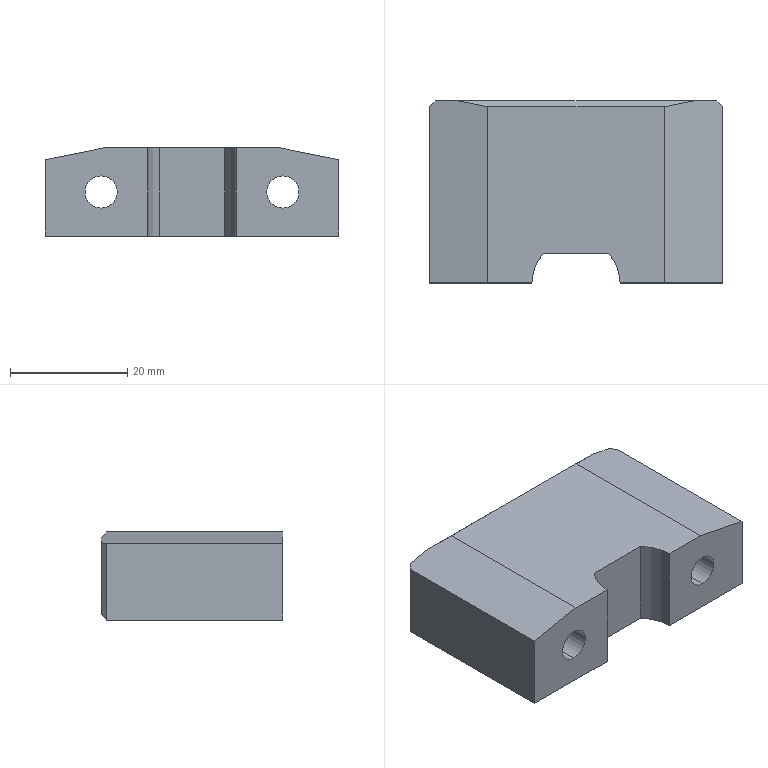Component | SolidWorks | XT-1-18-2-1 | 1 solid | 26 faces | box 50 x 31 x 15 mm | volume 18972 mm3 | plane 16 | cylinder 10 | commonest cylinder face diameters 10 x4 5.5 x4 15 x2
build123d program:
from build123d import *

# Parameters (mm, degrees)
BOSS_EXTRUDE1_DEPTH                             = 15
M5_HEX_SOCKET_HEAD_CAP_SCREW_CBORE1_D           = 5.5
M5_HEX_SOCKET_HEAD_CAP_SCREW_CBORE1_CBORE_D     = 10
M5_HEX_SOCKET_HEAD_CAP_SCREW_CBORE1_CBORE_DEPTH = 10
CHAMFER1_SIZE                                   = 10
CHAMFER1_SIZE2                                  = 2
CHAMFER2_SIZE                                   = 1
CHAMFER3_SIZE                                   = 1


with BuildPart() as part:
    # Sketch1 → Boss-Extrude1 (new body)
    with BuildSketch(Plane.XY):
        with BuildLine():
            Line((19.41, -26), (30.59, -26))
            ThreePointArc((30.59, -26), (32.006, -28.324), (32.5, -31))
            Line((32.5, -31), (50, -31))
            Line((50, -31), (50, 0))
            Line((50, 0), (0, 0))
            Line((0, 0), (0, -31))
            Line((0, -31), (17.5, -31))
            ThreePointArc((17.5, -31), (17.994, -28.324), (19.41, -26))
        make_face()
    extrude(amount=BOSS_EXTRUDE1_DEPTH)

    # M5 Hex Socket Head Cap Screw CBORE1 (through all)
    with Locations(Plane(origin=(0, 0, 0), x_dir=(1, 0, 0), z_dir=(0, 1, 0))):
        with Locations((9.5, -7.5), (40.5, -7.5)):
            CounterBoreHole(M5_HEX_SOCKET_HEAD_CAP_SCREW_CBORE1_D / 2, M5_HEX_SOCKET_HEAD_CAP_SCREW_CBORE1_CBORE_D / 2, M5_HEX_SOCKET_HEAD_CAP_SCREW_CBORE1_CBORE_DEPTH)

    # Chamfer1
    chamfer1_edges = [part.edges().sort_by_distance(p)[0] for p in [
        (0, -15.5, 0),
        (50, -15.5, 0),
    ]]
    chamfer1_side = [part.faces().sort_by_distance(p)[0] for p in [
        (25, -14.889, 0),
    ]]
    chamfer(chamfer1_edges, length=CHAMFER1_SIZE, length2=CHAMFER1_SIZE2, reference=chamfer1_side[0])

    # Chamfer2
    chamfer2_edges = [part.edges().sort_by_distance(p)[0] for p in [
        (25, 0, 15),
        (25, 0, 0),
    ]]
    chamfer(chamfer2_edges, length=CHAMFER2_SIZE)

    # Chamfer3
    chamfer3_edges = [part.edges().sort_by_distance(p)[0] for p in [
        (0, 0, 8),
        (50, 0, 8),
    ]]
    chamfer(chamfer3_edges, length=CHAMFER3_SIZE)


solid = part.part

# Placed as in the assembly
solid = solid.moved(Location((964.283, 139.385, -138), (-180, 0, 180)))
STEP:
#1=CARTESIAN_POINT('',(37.59,5.094,-5.531));
#2=VERTEX_POINT('',#1);
#3=CARTESIAN_POINT('',(37.59,5.094,-5.925));
#4=VERTEX_POINT('',#3);
#5=CARTESIAN_POINT('',(37.59,5.094,-5.728));
#6=DIRECTION('',(0.,1.,0.));
#7=DIRECTION('',(0.,0.,-1.));
#8=AXIS2_PLACEMENT_3D('',#5,#6,#7);
#9=CIRCLE('',#8,0.1969);
#10=EDGE_CURVE('',#2,#4,#9,.T.);
#11=ORIENTED_EDGE('',*,*,#10,.F.);
#12=CARTESIAN_POINT('',(37.59,5.488,-5.531));
#13=VERTEX_POINT('',#12);
#14=CARTESIAN_POINT('',(37.59,5.488,-5.531));
#15=DIRECTION('',(0.,1.,0.));
#16=VECTOR('',#15,39.37);
#17=LINE('',#14,#16);
#18=EDGE_CURVE('',#2,#13,#17,.T.);
#19=ORIENTED_EDGE('',*,*,#18,.T.);
#20=CARTESIAN_POINT('',(37.59,5.488,-5.925));
#21=VERTEX_POINT('',#20);
#22=CARTESIAN_POINT('',(37.59,5.488,-5.728));
#23=DIRECTION('',(0.,1.,0.));
#24=DIRECTION('',(0.,0.,-1.));
#25=AXIS2_PLACEMENT_3D('',#22,#23,#24);
#26=CIRCLE('',#25,0.1969);
#27=EDGE_CURVE('',#13,#21,#26,.T.);
#28=ORIENTED_EDGE('',*,*,#27,.T.);
#29=CARTESIAN_POINT('',(37.59,5.488,-5.925));
#30=DIRECTION('',(0.,1.,0.));
#31=VECTOR('',#30,39.37);
#32=LINE('',#29,#31);
#33=EDGE_CURVE('',#4,#21,#32,.T.);
#34=ORIENTED_EDGE('',*,*,#33,.F.);
#35=EDGE_LOOP('',(#11,#19,#28,#34));
#36=FACE_OUTER_BOUND('',#35,.T.);
#37=CARTESIAN_POINT('',(37.59,5.488,-5.728));
#38=DIRECTION('',(0.,1.,0.));
#39=DIRECTION('',(0.,0.,-1.));
#40=AXIS2_PLACEMENT_3D('',#37,#38,#39);
#41=CYLINDRICAL_SURFACE('',#40,0.1969);
#42=ADVANCED_FACE('',(#36),#41,.F.);
#43=CARTESIAN_POINT('',(37.59,4.267,-5.62));
#44=VERTEX_POINT('',#43);
#45=CARTESIAN_POINT('',(37.59,4.267,-5.837));
#46=VERTEX_POINT('',#45);
#47=CARTESIAN_POINT('',(37.59,4.267,-5.728));
#48=DIRECTION('',(0.,1.,0.));
#49=DIRECTION('',(0.,0.,-1.));
#50=AXIS2_PLACEMENT_3D('',#47,#48,#49);
#51=CIRCLE('',#50,0.1083);
#52=EDGE_CURVE('',#44,#46,#51,.T.);
#53=ORIENTED_EDGE('',*,*,#52,.F.);
#54=CARTESIAN_POINT('',(37.59,5.094,-5.62));
#55=VERTEX_POINT('',#54);
#56=CARTESIAN_POINT('',(37.59,5.488,-5.62));
#57=DIRECTION('',(0.,1.,0.));
#58=VECTOR('',#57,39.37);
#59=LINE('',#56,#58);
#60=EDGE_CURVE('',#44,#55,#59,.T.);
#61=ORIENTED_EDGE('',*,*,#60,.T.);
#62=CARTESIAN_POINT('',(37.59,5.094,-5.837));
#63=VERTEX_POINT('',#62);
#64=CARTESIAN_POINT('',(37.59,5.094,-5.728));
#65=DIRECTION('',(0.,1.,0.));
#66=DIRECTION('',(0.,0.,-1.));
#67=AXIS2_PLACEMENT_3D('',#64,#65,#66);
#68=CIRCLE('',#67,0.1083);
#69=EDGE_CURVE('',#55,#63,#68,.T.);
#70=ORIENTED_EDGE('',*,*,#69,.T.);
#71=CARTESIAN_POINT('',(37.59,5.488,-5.837));
#72=DIRECTION('',(0.,1.,0.));
#73=VECTOR('',#72,39.37);
#74=LINE('',#71,#73);
#75=EDGE_CURVE('',#46,#63,#74,.T.);
#76=ORIENTED_EDGE('',*,*,#75,.F.);
#77=EDGE_LOOP('',(#53,#61,#70,#76));
#78=FACE_OUTER_BOUND('',#77,.T.);
#79=CARTESIAN_POINT('',(37.59,5.488,-5.728));
#80=DIRECTION('',(0.,1.,0.));
#81=DIRECTION('',(0.,0.,-1.));
#82=AXIS2_PLACEMENT_3D('',#79,#80,#81);
#83=CYLINDRICAL_SURFACE('',#82,0.1083);
#84=ADVANCED_FACE('',(#78),#83,.F.);
#85=CARTESIAN_POINT('',(36.369,5.094,-5.531));
#86=VERTEX_POINT('',#85);
#87=CARTESIAN_POINT('',(36.369,5.094,-5.925));
#88=VERTEX_POINT('',#87);
#89=CARTESIAN_POINT('',(36.369,5.094,-5.728));
#90=DIRECTION('',(0.,1.,0.));
#91=DIRECTION('',(0.,0.,-1.));
#92=AXIS2_PLACEMENT_3D('',#89,#90,#91);
#93=CIRCLE('',#92,0.1969);
#94=EDGE_CURVE('',#86,#88,#93,.T.);
#95=ORIENTED_EDGE('',*,*,#94,.F.);
#96=CARTESIAN_POINT('',(36.369,5.488,-5.531));
#97=VERTEX_POINT('',#96);
#98=CARTESIAN_POINT('',(36.369,5.488,-5.531));
#99=DIRECTION('',(0.,1.,0.));
#100=VECTOR('',#99,39.37);
#101=LINE('',#98,#100);
#102=EDGE_CURVE('',#86,#97,#101,.T.);
#103=ORIENTED_EDGE('',*,*,#102,.T.);
#104=CARTESIAN_POINT('',(36.369,5.488,-5.925));
#105=VERTEX_POINT('',#104);
#106=CARTESIAN_POINT('',(36.369,5.488,-5.728));
#107=DIRECTION('',(0.,1.,0.));
#108=DIRECTION('',(0.,0.,-1.));
#109=AXIS2_PLACEMENT_3D('',#106,#107,#108);
#110=CIRCLE('',#109,0.1969);
#111=EDGE_CURVE('',#97,#105,#110,.T.);
#112=ORIENTED_EDGE('',*,*,#111,.T.);
#113=CARTESIAN_POINT('',(36.369,5.488,-5.925));
#114=DIRECTION('',(0.,1.,0.));
#115=VECTOR('',#114,39.37);
#116=LINE('',#113,#115);
#117=EDGE_CURVE('',#88,#105,#116,.T.);
#118=ORIENTED_EDGE('',*,*,#117,.F.);
#119=EDGE_LOOP('',(#95,#103,#112,#118));
#120=FACE_OUTER_BOUND('',#119,.T.);
#121=CARTESIAN_POINT('',(36.369,5.488,-5.728));
#122=DIRECTION('',(0.,1.,0.));
#123=DIRECTION('',(0.,0.,-1.));
#124=AXIS2_PLACEMENT_3D('',#121,#122,#123);
#125=CYLINDRICAL_SURFACE('',#124,0.1969);
#126=ADVANCED_FACE('',(#120),#125,.F.);
#127=CARTESIAN_POINT('',(36.369,4.267,-5.62));
#128=VERTEX_POINT('',#127);
#129=CARTESIAN_POINT('',(36.369,4.267,-5.837));
#130=VERTEX_POINT('',#129);
#131=CARTESIAN_POINT('',(36.369,4.267,-5.728));
#132=DIRECTION('',(0.,1.,0.));
#133=DIRECTION('',(0.,0.,-1.));
#134=AXIS2_PLACEMENT_3D('',#131,#132,#133);
#135=CIRCLE('',#134,0.1083);
#136=EDGE_CURVE('',#128,#130,#135,.T.);
#137=ORIENTED_EDGE('',*,*,#136,.F.);
#138=CARTESIAN_POINT('',(36.369,5.094,-5.62));
#139=VERTEX_POINT('',#138);
#140=CARTESIAN_POINT('',(36.369,5.488,-5.62));
#141=DIRECTION('',(0.,1.,0.));
#142=VECTOR('',#141,39.37);
#143=LINE('',#140,#142);
#144=EDGE_CURVE('',#128,#139,#143,.T.);
#145=ORIENTED_EDGE('',*,*,#144,.T.);
#146=CARTESIAN_POINT('',(36.369,5.094,-5.837));
#147=VERTEX_POINT('',#146);
#148=CARTESIAN_POINT('',(36.369,5.094,-5.728));
#149=DIRECTION('',(0.,1.,0.));
#150=DIRECTION('',(0.,0.,-1.));
#151=AXIS2_PLACEMENT_3D('',#148,#149,#150);
#152=CIRCLE('',#151,0.1083);
#153=EDGE_CURVE('',#139,#147,#152,.T.);
#154=ORIENTED_EDGE('',*,*,#153,.T.);
#155=CARTESIAN_POINT('',(36.369,5.488,-5.837));
#156=DIRECTION('',(0.,1.,0.));
#157=VECTOR('',#156,39.37);
#158=LINE('',#155,#157);
#159=EDGE_CURVE('',#130,#147,#158,.T.);
#160=ORIENTED_EDGE('',*,*,#159,.F.);
#161=EDGE_LOOP('',(#137,#145,#154,#160));
#162=FACE_OUTER_BOUND('',#161,.T.);
#163=CARTESIAN_POINT('',(36.369,5.488,-5.728));
#164=DIRECTION('',(0.,1.,0.));
#165=DIRECTION('',(0.,0.,-1.));
#166=AXIS2_PLACEMENT_3D('',#163,#164,#165);
#167=CYLINDRICAL_SURFACE('',#166,0.1083);
#168=ADVANCED_FACE('',(#162),#167,.F.);
#169=CARTESIAN_POINT('',(37.964,5.448,-6.024));
#170=VERTEX_POINT('',#169);
#171=CARTESIAN_POINT('',(37.964,4.267,-6.024));
#172=VERTEX_POINT('',#171);
#173=CARTESIAN_POINT('',(37.964,5.488,-6.024));
#174=DIRECTION('',(-0.,-1.,0.));
#175=VECTOR('',#174,39.37);
#176=LINE('',#173,#175);
#177=EDGE_CURVE('',#170,#172,#176,.T.);
#178=ORIENTED_EDGE('',*,*,#177,.F.);
#179=CARTESIAN_POINT('',(37.964,5.448,-5.512));
#180=VERTEX_POINT('',#179);
#181=CARTESIAN_POINT('',(37.964,5.448,-6.024));
#182=DIRECTION('',(0.,0.,1.));
#183=VECTOR('',#182,39.37);
#184=LINE('',#181,#183);
#185=EDGE_CURVE('',#170,#180,#184,.T.);
#186=ORIENTED_EDGE('',*,*,#185,.T.);
#187=CARTESIAN_POINT('',(37.964,4.267,-5.512));
#188=VERTEX_POINT('',#187);
#189=CARTESIAN_POINT('',(37.964,5.488,-5.512));
#190=DIRECTION('',(-0.,-1.,0.));
#191=VECTOR('',#190,39.37);
#192=LINE('',#189,#191);
#193=EDGE_CURVE('',#180,#188,#192,.T.);
#194=ORIENTED_EDGE('',*,*,#193,.T.);
#195=CARTESIAN_POINT('',(37.964,4.267,-6.024));
#196=DIRECTION('',(0.,0.,1.));
#197=VECTOR('',#196,39.37);
#198=LINE('',#195,#197);
#199=EDGE_CURVE('',#172,#188,#198,.T.);
#200=ORIENTED_EDGE('',*,*,#199,.F.);
#201=EDGE_LOOP('',(#178,#186,#194,#200));
#202=FACE_OUTER_BOUND('',#201,.T.);
#203=CARTESIAN_POINT('',(37.964,5.488,-6.024));
#204=DIRECTION('',(-1.,0.,0.));
#205=DIRECTION('',(0.,1.,0.));
#206=AXIS2_PLACEMENT_3D('',#203,#204,#205);
#207=PLANE('',#206);
#208=ADVANCED_FACE('',(#202),#207,.F.);
#209=CARTESIAN_POINT('',(37.59,4.267,-5.728));
#210=DIRECTION('',(0.,1.,0.));
#211=DIRECTION('',(0.,0.,-1.));
#212=AXIS2_PLACEMENT_3D('',#209,#210,#211);
#213=CIRCLE('',#212,0.1083);
#214=EDGE_CURVE('',#46,#44,#213,.T.);
#215=ORIENTED_EDGE('',*,*,#214,.T.);
#216=ORIENTED_EDGE('',*,*,#52,.T.);
#217=EDGE_LOOP('',(#215,#216));
#218=FACE_BOUND('',#217,.T.);
#219=ORIENTED_EDGE('',*,*,#199,.T.);
#220=CARTESIAN_POINT('',(37.57,4.267,-5.433));
#221=VERTEX_POINT('',#220);
#222=CARTESIAN_POINT('',(37.964,4.267,-5.512));
#223=DIRECTION('',(-0.9806,0.,0.1961));
#224=VECTOR('',#223,39.37);
#225=LINE('',#222,#224);
#226=EDGE_CURVE('',#188,#221,#225,.T.);
#227=ORIENTED_EDGE('',*,*,#226,.T.);
#228=CARTESIAN_POINT('',(37.275,4.267,-5.433));
#229=VERTEX_POINT('',#228);
#230=CARTESIAN_POINT('',(37.964,4.267,-5.433));
#231=DIRECTION('',(-1.,0.,0.));
#232=VECTOR('',#231,39.37);
#233=LINE('',#230,#232);
#234=EDGE_CURVE('',#221,#229,#233,.T.);
#235=ORIENTED_EDGE('',*,*,#234,.T.);
#236=CARTESIAN_POINT('',(37.275,4.267,-6.024));
#237=VERTEX_POINT('',#236);
#238=CARTESIAN_POINT('',(37.275,4.267,-6.024));
#239=DIRECTION('',(0.,0.,1.));
#240=VECTOR('',#239,39.37);
#241=LINE('',#238,#240);
#242=EDGE_CURVE('',#237,#229,#241,.T.);
#243=ORIENTED_EDGE('',*,*,#242,.F.);
#244=CARTESIAN_POINT('',(37.964,4.267,-6.024));
#245=DIRECTION('',(-1.,0.,0.));
#246=VECTOR('',#245,39.37);
#247=LINE('',#244,#246);
#248=EDGE_CURVE('',#172,#237,#247,.T.);
#249=ORIENTED_EDGE('',*,*,#248,.F.);
#250=EDGE_LOOP('',(#219,#227,#235,#243,#249));
#251=FACE_OUTER_BOUND('',#250,.T.);
#252=CARTESIAN_POINT('',(37.964,4.267,-6.024));
#253=DIRECTION('',(0.,1.,0.));
#254=DIRECTION('',(0.,0.,-1.));
#255=AXIS2_PLACEMENT_3D('',#252,#253,#254);
#256=PLANE('',#255);
#257=ADVANCED_FACE('',(#218,#251),#256,.F.);
#258=CARTESIAN_POINT('',(37.2,4.464,-5.433));
#259=VERTEX_POINT('',#258);
#260=CARTESIAN_POINT('',(36.98,4.267,-5.433));
#261=DIRECTION('',(0.,0.,1.));
#262=DIRECTION('',(-1.,0.,0.));
#263=AXIS2_PLACEMENT_3D('',#260,#261,#262);
#264=CIRCLE('',#263,0.2953);
#265=EDGE_CURVE('',#229,#259,#264,.T.);
#266=ORIENTED_EDGE('',*,*,#265,.T.);
#267=CARTESIAN_POINT('',(37.2,4.464,-6.024));
#268=VERTEX_POINT('',#267);
#269=CARTESIAN_POINT('',(37.2,4.464,-6.024));
#270=DIRECTION('',(0.,0.,1.));
#271=VECTOR('',#270,39.37);
#272=LINE('',#269,#271);
#273=EDGE_CURVE('',#268,#259,#272,.T.);
#274=ORIENTED_EDGE('',*,*,#273,.F.);
#275=CARTESIAN_POINT('',(36.98,4.267,-6.024));
#276=DIRECTION('',(0.,0.,1.));
#277=DIRECTION('',(-1.,0.,0.));
#278=AXIS2_PLACEMENT_3D('',#275,#276,#277);
#279=CIRCLE('',#278,0.2953);
#280=EDGE_CURVE('',#237,#268,#279,.T.);
#281=ORIENTED_EDGE('',*,*,#280,.F.);
#282=ORIENTED_EDGE('',*,*,#242,.T.);
#283=EDGE_LOOP('',(#266,#274,#281,#282));
#284=FACE_OUTER_BOUND('',#283,.T.);
#285=CARTESIAN_POINT('',(36.98,4.267,-6.024));
#286=DIRECTION('',(0.,0.,1.));
#287=DIRECTION('',(1.,0.,0.));
#288=AXIS2_PLACEMENT_3D('',#285,#286,#287);
#289=CYLINDRICAL_SURFACE('',#288,0.2953);
#290=ADVANCED_FACE('',(#284),#289,.F.);
#291=CARTESIAN_POINT('',(36.76,4.464,-5.433));
#292=VERTEX_POINT('',#291);
#293=CARTESIAN_POINT('',(37.2,4.464,-5.433));
#294=DIRECTION('',(-1.,0.,0.));
#295=VECTOR('',#294,39.37);
#296=LINE('',#293,#295);
#297=EDGE_CURVE('',#259,#292,#296,.T.);
#298=ORIENTED_EDGE('',*,*,#297,.T.);
#299=CARTESIAN_POINT('',(36.76,4.464,-6.024));
#300=VERTEX_POINT('',#299);
#301=CARTESIAN_POINT('',(36.76,4.464,-6.024));
#302=DIRECTION('',(0.,0.,1.));
#303=VECTOR('',#302,39.37);
#304=LINE('',#301,#303);
#305=EDGE_CURVE('',#300,#292,#304,.T.);
#306=ORIENTED_EDGE('',*,*,#305,.F.);
#307=CARTESIAN_POINT('',(37.2,4.464,-6.024));
#308=DIRECTION('',(-1.,0.,0.));
#309=VECTOR('',#308,39.37);
#310=LINE('',#307,#309);
#311=EDGE_CURVE('',#268,#300,#310,.T.);
#312=ORIENTED_EDGE('',*,*,#311,.F.);
#313=ORIENTED_EDGE('',*,*,#273,.T.);
#314=EDGE_LOOP('',(#298,#306,#312,#313));
#315=FACE_OUTER_BOUND('',#314,.T.);
#316=CARTESIAN_POINT('',(37.2,4.464,-6.024));
#317=DIRECTION('',(0.,1.,0.));
#318=DIRECTION('',(0.,0.,-1.));
#319=AXIS2_PLACEMENT_3D('',#316,#317,#318);
#320=PLANE('',#319);
#321=ADVANCED_FACE('',(#315),#320,.F.);
#322=CARTESIAN_POINT('',(36.684,4.267,-5.433));
#323=VERTEX_POINT('',#322);
#324=CARTESIAN_POINT('',(36.98,4.267,-5.433));
#325=DIRECTION('',(0.,0.,1.));
#326=DIRECTION('',(-1.,0.,0.));
#327=AXIS2_PLACEMENT_3D('',#324,#325,#326);
#328=CIRCLE('',#327,0.2953);
#329=EDGE_CURVE('',#292,#323,#328,.T.);
#330=ORIENTED_EDGE('',*,*,#329,.T.);
#331=CARTESIAN_POINT('',(36.684,4.267,-6.024));
#332=VERTEX_POINT('',#331);
#333=CARTESIAN_POINT('',(36.684,4.267,-6.024));
#334=DIRECTION('',(0.,0.,1.));
#335=VECTOR('',#334,39.37);
#336=LINE('',#333,#335);
#337=EDGE_CURVE('',#332,#323,#336,.T.);
#338=ORIENTED_EDGE('',*,*,#337,.F.);
#339=CARTESIAN_POINT('',(36.98,4.267,-6.024));
#340=DIRECTION('',(0.,0.,1.));
#341=DIRECTION('',(-1.,0.,0.));
#342=AXIS2_PLACEMENT_3D('',#339,#340,#341);
#343=CIRCLE('',#342,0.2953);
#344=EDGE_CURVE('',#300,#332,#343,.T.);
#345=ORIENTED_EDGE('',*,*,#344,.F.);
#346=ORIENTED_EDGE('',*,*,#305,.T.);
#347=EDGE_LOOP('',(#330,#338,#345,#346));
#348=FACE_OUTER_BOUND('',#347,.T.);
#349=CARTESIAN_POINT('',(36.98,4.267,-6.024));
#350=DIRECTION('',(0.,0.,1.));
#351=DIRECTION('',(1.,0.,0.));
#352=AXIS2_PLACEMENT_3D('',#349,#350,#351);
#353=CYLINDRICAL_SURFACE('',#352,0.2953);
#354=ADVANCED_FACE('',(#348),#353,.F.);
#355=CARTESIAN_POINT('',(36.369,4.267,-5.728));
#356=DIRECTION('',(0.,1.,0.));
#357=DIRECTION('',(0.,0.,-1.));
#358=AXIS2_PLACEMENT_3D('',#355,#356,#357);
#359=CIRCLE('',#358,0.1083);
#360=EDGE_CURVE('',#130,#128,#359,.T.);
#361=ORIENTED_EDGE('',*,*,#360,.T.);
#362=ORIENTED_EDGE('',*,*,#136,.T.);
#363=EDGE_LOOP('',(#361,#362));
#364=FACE_BOUND('',#363,.T.);
#365=CARTESIAN_POINT('',(36.389,4.267,-5.433));
#366=VERTEX_POINT('',#365);
#367=CARTESIAN_POINT('',(36.684,4.267,-5.433));
#368=DIRECTION('',(-1.,0.,0.));
#369=VECTOR('',#368,39.37);
#370=LINE('',#367,#369);
#371=EDGE_CURVE('',#323,#366,#370,.T.);
#372=ORIENTED_EDGE('',*,*,#371,.T.);
#373=CARTESIAN_POINT('',(35.995,4.267,-5.512));
#374=VERTEX_POINT('',#373);
#375=CARTESIAN_POINT('',(35.995,4.267,-5.512));
#376=DIRECTION('',(-0.9806,0.,-0.1961));
#377=VECTOR('',#376,39.37);
#378=LINE('',#375,#377);
#379=EDGE_CURVE('',#366,#374,#378,.T.);
#380=ORIENTED_EDGE('',*,*,#379,.T.);
#381=CARTESIAN_POINT('',(35.995,4.267,-6.024));
#382=VERTEX_POINT('',#381);
#383=CARTESIAN_POINT('',(35.995,4.267,-6.024));
#384=DIRECTION('',(0.,0.,1.));
#385=VECTOR('',#384,39.37);
#386=LINE('',#383,#385);
#387=EDGE_CURVE('',#382,#374,#386,.T.);
#388=ORIENTED_EDGE('',*,*,#387,.F.);
#389=CARTESIAN_POINT('',(36.684,4.267,-6.024));
#390=DIRECTION('',(-1.,0.,0.));
#391=VECTOR('',#390,39.37);
#392=LINE('',#389,#391);
#393=EDGE_CURVE('',#332,#382,#392,.T.);
#394=ORIENTED_EDGE('',*,*,#393,.F.);
#395=ORIENTED_EDGE('',*,*,#337,.T.);
#396=EDGE_LOOP('',(#372,#380,#388,#394,#395));
#397=FACE_OUTER_BOUND('',#396,.T.);
#398=CARTESIAN_POINT('',(36.684,4.267,-6.024));
#399=DIRECTION('',(0.,1.,0.));
#400=DIRECTION('',(1.,-0.,0.));
#401=AXIS2_PLACEMENT_3D('',#398,#399,#400);
#402=PLANE('',#401);
#403=ADVANCED_FACE('',(#364,#397),#402,.F.);
#404=CARTESIAN_POINT('',(35.995,5.448,-5.512));
#405=VERTEX_POINT('',#404);
#406=CARTESIAN_POINT('',(35.995,5.488,-5.512));
#407=DIRECTION('',(0.,1.,0.));
#408=VECTOR('',#407,39.37);
#409=LINE('',#406,#408);
#410=EDGE_CURVE('',#374,#405,#409,.T.);
#411=ORIENTED_EDGE('',*,*,#410,.T.);
#412=CARTESIAN_POINT('',(35.995,5.448,-6.024));
#413=VERTEX_POINT('',#412);
#414=CARTESIAN_POINT('',(35.995,5.448,-6.024));
#415=DIRECTION('',(0.,0.,-1.));
#416=VECTOR('',#415,39.37);
#417=LINE('',#414,#416);
#418=EDGE_CURVE('',#405,#413,#417,.T.);
#419=ORIENTED_EDGE('',*,*,#418,.T.);
#420=CARTESIAN_POINT('',(35.995,5.488,-6.024));
#421=DIRECTION('',(0.,1.,0.));
#422=VECTOR('',#421,39.37);
#423=LINE('',#420,#422);
#424=EDGE_CURVE('',#382,#413,#423,.T.);
#425=ORIENTED_EDGE('',*,*,#424,.F.);
#426=ORIENTED_EDGE('',*,*,#387,.T.);
#427=EDGE_LOOP('',(#411,#419,#425,#426));
#428=FACE_OUTER_BOUND('',#427,.T.);
#429=CARTESIAN_POINT('',(35.995,5.488,-6.024));
#430=DIRECTION('',(1.,-0.,0.));
#431=DIRECTION('',(-0.,-1.,0.));
#432=AXIS2_PLACEMENT_3D('',#429,#430,#431);
#433=PLANE('',#432);
#434=ADVANCED_FACE('',(#428),#433,.F.);
#435=CARTESIAN_POINT('',(37.59,5.488,-5.728));
#436=DIRECTION('',(0.,1.,0.));
#437=DIRECTION('',(0.,0.,-1.));
#438=AXIS2_PLACEMENT_3D('',#435,#436,#437);
#439=CIRCLE('',#438,0.1969);
#440=EDGE_CURVE('',#21,#13,#439,.T.);
#441=ORIENTED_EDGE('',*,*,#440,.F.);
#442=ORIENTED_EDGE('',*,*,#27,.F.);
#443=EDGE_LOOP('',(#441,#442));
#444=FACE_BOUND('',#443,.T.);
#445=CARTESIAN_POINT('',(36.369,5.488,-5.728));
#446=DIRECTION('',(0.,1.,0.));
#447=DIRECTION('',(0.,0.,-1.));
#448=AXIS2_PLACEMENT_3D('',#445,#446,#447);
#449=CIRCLE('',#448,0.1969);
#450=EDGE_CURVE('',#105,#97,#449,.T.);
#451=ORIENTED_EDGE('',*,*,#450,.F.);
#452=ORIENTED_EDGE('',*,*,#111,.F.);
#453=EDGE_LOOP('',(#451,#452));
#454=FACE_BOUND('',#453,.T.);
#455=CARTESIAN_POINT('',(37.767,5.488,-5.472));
#456=VERTEX_POINT('',#455);
#457=CARTESIAN_POINT('',(37.925,5.488,-5.504));
#458=VERTEX_POINT('',#457);
#459=CARTESIAN_POINT('',(37.964,5.488,-5.512));
#460=DIRECTION('',(0.9806,0.,-0.1961));
#461=VECTOR('',#460,39.37);
#462=LINE('',#459,#461);
#463=EDGE_CURVE('',#456,#458,#462,.T.);
#464=ORIENTED_EDGE('',*,*,#463,.T.);
#465=CARTESIAN_POINT('',(37.925,5.488,-5.984));
#466=VERTEX_POINT('',#465);
#467=CARTESIAN_POINT('',(37.925,5.488,-6.024));
#468=DIRECTION('',(0.,0.,-1.));
#469=VECTOR('',#468,39.37);
#470=LINE('',#467,#469);
#471=EDGE_CURVE('',#458,#466,#470,.T.);
#472=ORIENTED_EDGE('',*,*,#471,.T.);
#473=CARTESIAN_POINT('',(36.035,5.488,-5.984));
#474=VERTEX_POINT('',#473);
#475=CARTESIAN_POINT('',(35.995,5.488,-5.984));
#476=DIRECTION('',(-1.,0.,0.));
#477=VECTOR('',#476,39.37);
#478=LINE('',#475,#477);
#479=EDGE_CURVE('',#466,#474,#478,.T.);
#480=ORIENTED_EDGE('',*,*,#479,.T.);
#481=CARTESIAN_POINT('',(36.035,5.488,-5.504));
#482=VERTEX_POINT('',#481);
#483=CARTESIAN_POINT('',(36.035,5.488,-6.024));
#484=DIRECTION('',(0.,0.,1.));
#485=VECTOR('',#484,39.37);
#486=LINE('',#483,#485);
#487=EDGE_CURVE('',#474,#482,#486,.T.);
#488=ORIENTED_EDGE('',*,*,#487,.T.);
#489=CARTESIAN_POINT('',(36.192,5.488,-5.472));
#490=VERTEX_POINT('',#489);
#491=CARTESIAN_POINT('',(35.995,5.488,-5.512));
#492=DIRECTION('',(0.9806,0.,0.1961));
#493=VECTOR('',#492,39.37);
#494=LINE('',#491,#493);
#495=EDGE_CURVE('',#482,#490,#494,.T.);
#496=ORIENTED_EDGE('',*,*,#495,.T.);
#497=CARTESIAN_POINT('',(37.964,5.488,-5.472));
#498=DIRECTION('',(1.,0.,0.));
#499=VECTOR('',#498,39.37);
#500=LINE('',#497,#499);
#501=EDGE_CURVE('',#490,#456,#500,.T.);
#502=ORIENTED_EDGE('',*,*,#501,.T.);
#503=EDGE_LOOP('',(#464,#472,#480,#488,#496,#502));
#504=FACE_OUTER_BOUND('',#503,.T.);
#505=CARTESIAN_POINT('',(37.964,5.488,-6.024));
#506=DIRECTION('',(0.,-1.,0.));
#507=DIRECTION('',(0.,0.,1.));
#508=AXIS2_PLACEMENT_3D('',#505,#506,#507);
#509=PLANE('',#508);
#510=ADVANCED_FACE('',(#444,#454,#504),#509,.F.);
#511=ORIENTED_EDGE('',*,*,#424,.T.);
#512=CARTESIAN_POINT('',(37.964,5.448,-6.024));
#513=DIRECTION('',(1.,0.,0.));
#514=VECTOR('',#513,39.37);
#515=LINE('',#512,#514);
#516=EDGE_CURVE('',#413,#170,#515,.T.);
#517=ORIENTED_EDGE('',*,*,#516,.T.);
#518=ORIENTED_EDGE('',*,*,#177,.T.);
#519=ORIENTED_EDGE('',*,*,#248,.T.);
#520=ORIENTED_EDGE('',*,*,#280,.T.);
#521=ORIENTED_EDGE('',*,*,#311,.T.);
#522=ORIENTED_EDGE('',*,*,#344,.T.);
#523=ORIENTED_EDGE('',*,*,#393,.T.);
#524=EDGE_LOOP('',(#511,#517,#518,#519,#520,#521,#522,#523));
#525=FACE_OUTER_BOUND('',#524,.T.);
#526=CARTESIAN_POINT('',(36.98,4.267,-6.024));
#527=DIRECTION('',(0.,0.,-1.));
#528=DIRECTION('',(-1.,0.,0.));
#529=AXIS2_PLACEMENT_3D('',#526,#527,#528);
#530=PLANE('',#529);
#531=ADVANCED_FACE('',(#525),#530,.T.);
#532=CARTESIAN_POINT('',(37.57,5.448,-5.433));
#533=VERTEX_POINT('',#532);
#534=CARTESIAN_POINT('',(37.57,4.267,-5.433));
#535=DIRECTION('',(0.,1.,0.));
#536=VECTOR('',#535,39.37);
#537=LINE('',#534,#536);
#538=EDGE_CURVE('',#221,#533,#537,.T.);
#539=ORIENTED_EDGE('',*,*,#538,.T.);
#540=CARTESIAN_POINT('',(36.389,5.448,-5.433));
#541=VERTEX_POINT('',#540);
#542=CARTESIAN_POINT('',(36.98,5.448,-5.433));
#543=DIRECTION('',(-1.,0.,0.));
#544=VECTOR('',#543,39.37);
#545=LINE('',#542,#544);
#546=EDGE_CURVE('',#533,#541,#545,.T.);
#547=ORIENTED_EDGE('',*,*,#546,.T.);
#548=CARTESIAN_POINT('',(36.389,4.267,-5.433));
#549=DIRECTION('',(-0.,-1.,0.));
#550=VECTOR('',#549,39.37);
#551=LINE('',#548,#550);
#552=EDGE_CURVE('',#541,#366,#551,.T.);
#553=ORIENTED_EDGE('',*,*,#552,.T.);
#554=ORIENTED_EDGE('',*,*,#371,.F.);
#555=ORIENTED_EDGE('',*,*,#329,.F.);
#556=ORIENTED_EDGE('',*,*,#297,.F.);
#557=ORIENTED_EDGE('',*,*,#265,.F.);
#558=ORIENTED_EDGE('',*,*,#234,.F.);
#559=EDGE_LOOP('',(#539,#547,#553,#554,#555,#556,#557,#558));
#560=FACE_OUTER_BOUND('',#559,.T.);
#561=CARTESIAN_POINT('',(36.98,4.267,-5.433));
#562=DIRECTION('',(0.,0.,-1.));
#563=DIRECTION('',(-1.,0.,0.));
#564=AXIS2_PLACEMENT_3D('',#561,#562,#563);
#565=PLANE('',#564);
#566=ADVANCED_FACE('',(#560),#565,.F.);
#567=ORIENTED_EDGE('',*,*,#144,.F.);
#568=ORIENTED_EDGE('',*,*,#360,.F.);
#569=ORIENTED_EDGE('',*,*,#159,.T.);
#570=CARTESIAN_POINT('',(36.369,5.094,-5.728));
#571=DIRECTION('',(0.,1.,0.));
#572=DIRECTION('',(0.,0.,-1.));
#573=AXIS2_PLACEMENT_3D('',#570,#571,#572);
#574=CIRCLE('',#573,0.1083);
#575=EDGE_CURVE('',#147,#139,#574,.T.);
#576=ORIENTED_EDGE('',*,*,#575,.T.);
#577=EDGE_LOOP('',(#567,#568,#569,#576));
#578=FACE_OUTER_BOUND('',#577,.T.);
#579=CARTESIAN_POINT('',(36.369,5.488,-5.728));
#580=DIRECTION('',(0.,1.,0.));
#581=DIRECTION('',(0.,0.,-1.));
#582=AXIS2_PLACEMENT_3D('',#579,#580,#581);
#583=CYLINDRICAL_SURFACE('',#582,0.1083);
#584=ADVANCED_FACE('',(#578),#583,.F.);
#585=ORIENTED_EDGE('',*,*,#575,.F.);
#586=ORIENTED_EDGE('',*,*,#153,.F.);
#587=EDGE_LOOP('',(#585,#586));
#588=FACE_BOUND('',#587,.T.);
#589=CARTESIAN_POINT('',(36.369,5.094,-5.728));
#590=DIRECTION('',(0.,1.,0.));
#591=DIRECTION('',(0.,0.,-1.));
#592=AXIS2_PLACEMENT_3D('',#589,#590,#591);
#593=CIRCLE('',#592,0.1969);
#594=EDGE_CURVE('',#88,#86,#593,.T.);
#595=ORIENTED_EDGE('',*,*,#594,.T.);
#596=ORIENTED_EDGE('',*,*,#94,.T.);
#597=EDGE_LOOP('',(#595,#596));
#598=FACE_OUTER_BOUND('',#597,.T.);
#599=CARTESIAN_POINT('',(36.261,5.094,-5.728));
#600=DIRECTION('',(0.,-1.,0.));
#601=DIRECTION('',(0.,0.,1.));
#602=AXIS2_PLACEMENT_3D('',#599,#600,#601);
#603=PLANE('',#602);
#604=ADVANCED_FACE('',(#588,#598),#603,.F.);
#605=ORIENTED_EDGE('',*,*,#102,.F.);
#606=ORIENTED_EDGE('',*,*,#594,.F.);
#607=ORIENTED_EDGE('',*,*,#117,.T.);
#608=ORIENTED_EDGE('',*,*,#450,.T.);
#609=EDGE_LOOP('',(#605,#606,#607,#608));
#610=FACE_OUTER_BOUND('',#609,.T.);
#611=CARTESIAN_POINT('',(36.369,5.488,-5.728));
#612=DIRECTION('',(0.,1.,0.));
#613=DIRECTION('',(0.,0.,-1.));
#614=AXIS2_PLACEMENT_3D('',#611,#612,#613);
#615=CYLINDRICAL_SURFACE('',#614,0.1969);
#616=ADVANCED_FACE('',(#610),#615,.F.);
#617=ORIENTED_EDGE('',*,*,#60,.F.);
#618=ORIENTED_EDGE('',*,*,#214,.F.);
#619=ORIENTED_EDGE('',*,*,#75,.T.);
#620=CARTESIAN_POINT('',(37.59,5.094,-5.728));
#621=DIRECTION('',(0.,1.,0.));
#622=DIRECTION('',(0.,0.,-1.));
#623=AXIS2_PLACEMENT_3D('',#620,#621,#622);
#624=CIRCLE('',#623,0.1083);
#625=EDGE_CURVE('',#63,#55,#624,.T.);
#626=ORIENTED_EDGE('',*,*,#625,.T.);
#627=EDGE_LOOP('',(#617,#618,#619,#626));
#628=FACE_OUTER_BOUND('',#627,.T.);
#629=CARTESIAN_POINT('',(37.59,5.488,-5.728));
#630=DIRECTION('',(0.,1.,0.));
#631=DIRECTION('',(0.,0.,-1.));
#632=AXIS2_PLACEMENT_3D('',#629,#630,#631);
#633=CYLINDRICAL_SURFACE('',#632,0.1083);
#634=ADVANCED_FACE('',(#628),#633,.F.);
#635=ORIENTED_EDGE('',*,*,#625,.F.);
#636=ORIENTED_EDGE('',*,*,#69,.F.);
#637=EDGE_LOOP('',(#635,#636));
#638=FACE_BOUND('',#637,.T.);
#639=CARTESIAN_POINT('',(37.59,5.094,-5.728));
#640=DIRECTION('',(0.,1.,0.));
#641=DIRECTION('',(0.,0.,-1.));
#642=AXIS2_PLACEMENT_3D('',#639,#640,#641);
#643=CIRCLE('',#642,0.1969);
#644=EDGE_CURVE('',#4,#2,#643,.T.);
#645=ORIENTED_EDGE('',*,*,#644,.T.);
#646=ORIENTED_EDGE('',*,*,#10,.T.);
#647=EDGE_LOOP('',(#645,#646));
#648=FACE_OUTER_BOUND('',#647,.T.);
#649=CARTESIAN_POINT('',(37.482,5.094,-5.728));
#650=DIRECTION('',(0.,-1.,0.));
#651=DIRECTION('',(0.,0.,1.));
#652=AXIS2_PLACEMENT_3D('',#649,#650,#651);
#653=PLANE('',#652);
#654=ADVANCED_FACE('',(#638,#648),#653,.F.);
#655=ORIENTED_EDGE('',*,*,#18,.F.);
#656=ORIENTED_EDGE('',*,*,#644,.F.);
#657=ORIENTED_EDGE('',*,*,#33,.T.);
#658=ORIENTED_EDGE('',*,*,#440,.T.);
#659=EDGE_LOOP('',(#655,#656,#657,#658));
#660=FACE_OUTER_BOUND('',#659,.T.);
#661=CARTESIAN_POINT('',(37.59,5.488,-5.728));
#662=DIRECTION('',(0.,1.,0.));
#663=DIRECTION('',(0.,0.,-1.));
#664=AXIS2_PLACEMENT_3D('',#661,#662,#663);
#665=CYLINDRICAL_SURFACE('',#664,0.1969);
#666=ADVANCED_FACE('',(#660),#665,.F.);
#667=ORIENTED_EDGE('',*,*,#495,.F.);
#668=CARTESIAN_POINT('',(36.015,5.468,-5.508));
#669=DIRECTION('',(-0.7001,-0.7001,-0.14));
#670=VECTOR('',#669,39.37);
#671=LINE('',#668,#670);
#672=EDGE_CURVE('',#482,#405,#671,.T.);
#673=ORIENTED_EDGE('',*,*,#672,.T.);
#674=ORIENTED_EDGE('',*,*,#410,.F.);
#675=ORIENTED_EDGE('',*,*,#379,.F.);
#676=ORIENTED_EDGE('',*,*,#552,.F.);
#677=CARTESIAN_POINT('',(36.003,5.526,-5.51));
#678=DIRECTION('',(-0.9623,0.1925,-0.1925));
#679=VECTOR('',#678,39.37);
#680=LINE('',#677,#679);
#681=EDGE_CURVE('',#541,#490,#680,.T.);
#682=ORIENTED_EDGE('',*,*,#681,.T.);
#683=EDGE_LOOP('',(#667,#673,#674,#675,#676,#682));
#684=FACE_OUTER_BOUND('',#683,.T.);
#685=CARTESIAN_POINT('',(35.995,5.488,-5.512));
#686=DIRECTION('',(0.1961,-0.,-0.9806));
#687=DIRECTION('',(0.,1.,0.));
#688=AXIS2_PLACEMENT_3D('',#685,#686,#687);
#689=PLANE('',#688);
#690=ADVANCED_FACE('',(#684),#689,.F.);
#691=ORIENTED_EDGE('',*,*,#193,.F.);
#692=CARTESIAN_POINT('',(37.945,5.468,-5.508));
#693=DIRECTION('',(-0.7001,0.7001,0.14));
#694=VECTOR('',#693,39.37);
#695=LINE('',#692,#694);
#696=EDGE_CURVE('',#180,#458,#695,.T.);
#697=ORIENTED_EDGE('',*,*,#696,.T.);
#698=ORIENTED_EDGE('',*,*,#463,.F.);
#699=CARTESIAN_POINT('',(37.957,5.526,-5.51));
#700=DIRECTION('',(-0.9623,-0.1925,0.1925));
#701=VECTOR('',#700,39.37);
#702=LINE('',#699,#701);
#703=EDGE_CURVE('',#456,#533,#702,.T.);
#704=ORIENTED_EDGE('',*,*,#703,.T.);
#705=ORIENTED_EDGE('',*,*,#538,.F.);
#706=ORIENTED_EDGE('',*,*,#226,.F.);
#707=EDGE_LOOP('',(#691,#697,#698,#704,#705,#706));
#708=FACE_OUTER_BOUND('',#707,.T.);
#709=CARTESIAN_POINT('',(37.964,5.488,-5.512));
#710=DIRECTION('',(-0.1961,0.,-0.9806));
#711=DIRECTION('',(-0.,-1.,0.));
#712=AXIS2_PLACEMENT_3D('',#709,#710,#711);
#713=PLANE('',#712);
#714=ADVANCED_FACE('',(#708),#713,.F.);
#715=ORIENTED_EDGE('',*,*,#479,.F.);
#716=CARTESIAN_POINT('',(37.636,5.776,-5.696));
#717=DIRECTION('',(0.5774,-0.5774,-0.5774));
#718=VECTOR('',#717,39.37);
#719=LINE('',#716,#718);
#720=EDGE_CURVE('',#466,#170,#719,.T.);
#721=ORIENTED_EDGE('',*,*,#720,.T.);
#722=ORIENTED_EDGE('',*,*,#516,.F.);
#723=CARTESIAN_POINT('',(36.323,5.776,-5.696));
#724=DIRECTION('',(0.5774,0.5774,0.5774));
#725=VECTOR('',#724,39.37);
#726=LINE('',#723,#725);
#727=EDGE_CURVE('',#413,#474,#726,.T.);
#728=ORIENTED_EDGE('',*,*,#727,.T.);
#729=EDGE_LOOP('',(#715,#721,#722,#728));
#730=FACE_OUTER_BOUND('',#729,.T.);
#731=CARTESIAN_POINT('',(36.98,5.448,-6.024));
#732=DIRECTION('',(0.,0.7071,-0.7071));
#733=DIRECTION('',(-1.,0.,0.));
#734=AXIS2_PLACEMENT_3D('',#731,#732,#733);
#735=PLANE('',#734);
#736=ADVANCED_FACE('',(#730),#735,.T.);
#737=ORIENTED_EDGE('',*,*,#681,.F.);
#738=ORIENTED_EDGE('',*,*,#546,.F.);
#739=ORIENTED_EDGE('',*,*,#703,.F.);
#740=ORIENTED_EDGE('',*,*,#501,.F.);
#741=EDGE_LOOP('',(#737,#738,#739,#740));
#742=FACE_OUTER_BOUND('',#741,.T.);
#743=CARTESIAN_POINT('',(37.964,5.488,-5.472));
#744=DIRECTION('',(0.,-0.7071,-0.7071));
#745=DIRECTION('',(1.,0.,0.));
#746=AXIS2_PLACEMENT_3D('',#743,#744,#745);
#747=PLANE('',#746);
#748=ADVANCED_FACE('',(#742),#747,.F.);
#749=ORIENTED_EDGE('',*,*,#720,.F.);
#750=ORIENTED_EDGE('',*,*,#471,.F.);
#751=ORIENTED_EDGE('',*,*,#696,.F.);
#752=ORIENTED_EDGE('',*,*,#185,.F.);
#753=EDGE_LOOP('',(#749,#750,#751,#752));
#754=FACE_OUTER_BOUND('',#753,.T.);
#755=CARTESIAN_POINT('',(37.964,5.448,-6.024));
#756=DIRECTION('',(-0.7071,-0.7071,0.));
#757=DIRECTION('',(0.,0.,1.));
#758=AXIS2_PLACEMENT_3D('',#755,#756,#757);
#759=PLANE('',#758);
#760=ADVANCED_FACE('',(#754),#759,.F.);
#761=ORIENTED_EDGE('',*,*,#727,.F.);
#762=ORIENTED_EDGE('',*,*,#418,.F.);
#763=ORIENTED_EDGE('',*,*,#672,.F.);
#764=ORIENTED_EDGE('',*,*,#487,.F.);
#765=EDGE_LOOP('',(#761,#762,#763,#764));
#766=FACE_OUTER_BOUND('',#765,.T.);
#767=CARTESIAN_POINT('',(36.035,5.488,-6.024));
#768=DIRECTION('',(0.7071,-0.7071,0.));
#769=DIRECTION('',(0.,0.,1.));
#770=AXIS2_PLACEMENT_3D('',#767,#768,#769);
#771=PLANE('',#770);
#772=ADVANCED_FACE('',(#766),#771,.F.);
#773=CLOSED_SHELL('',(#42,#84,#126,#168,#208,#257,#290,#321,#354,#403,#434,#510,#531,#566,#584,#604,#616,#634,#654,#666,#690,#714,#736,#748,#760,#772));
#774=MANIFOLD_SOLID_BREP('',#773);
#775=CARTESIAN_POINT('',(0.,0.,0.));
#776=DIRECTION('',(0.,0.,1.));
#777=DIRECTION('',(1.,0.,0.));
#778=AXIS2_PLACEMENT_3D('',#775,#776,#777);
#779=(LENGTH_UNIT()NAMED_UNIT(*)SI_UNIT($,.METRE.));
#780=LENGTH_MEASURE_WITH_UNIT(LENGTH_MEASURE(0.0254),#779);
#781=DIMENSIONAL_EXPONENTS(1.,0.,0.,0.,0.,0.,0.);
#782=(CONVERSION_BASED_UNIT('',#780)LENGTH_UNIT()NAMED_UNIT(#781));
#783=UNCERTAINTY_MEASURE_WITH_UNIT(LENGTH_MEASURE(0.00001),#782,'','');
#784=(NAMED_UNIT(*)PLANE_ANGLE_UNIT()SI_UNIT($,.RADIAN.));
#785=(NAMED_UNIT(*)SI_UNIT($,.STERADIAN.)SOLID_ANGLE_UNIT());
#786=(GEOMETRIC_REPRESENTATION_CONTEXT(3)GLOBAL_UNCERTAINTY_ASSIGNED_CONTEXT((#783))GLOBAL_UNIT_ASSIGNED_CONTEXT((#782,#784,#785))REPRESENTATION_CONTEXT('',''));
#787=ADVANCED_BREP_SHAPE_REPRESENTATION('',(#774,#778),#786);
#788=COLOUR_RGB('',0.7922,0.8196,0.9333);
#789=FILL_AREA_STYLE_COLOUR('',#788);
#790=FILL_AREA_STYLE('',(#789));
#791=SURFACE_STYLE_FILL_AREA(#790);
#792=SURFACE_SIDE_STYLE('',(#791));
#793=SURFACE_STYLE_USAGE(.BOTH.,#792);
#794=PRESENTATION_STYLE_ASSIGNMENT((#793));
#795=STYLED_ITEM('',(#794),#774);
#796=PRESENTATION_LAYER_ASSIGNMENT('','',(#795));
#797=(LENGTH_UNIT()NAMED_UNIT(*)SI_UNIT($,.METRE.));
#798=LENGTH_MEASURE_WITH_UNIT(LENGTH_MEASURE(0.0254),#797);
#799=DIMENSIONAL_EXPONENTS(1.,0.,0.,0.,0.,0.,0.);
#800=(CONVERSION_BASED_UNIT('',#798)LENGTH_UNIT()NAMED_UNIT(#799));
#801=UNCERTAINTY_MEASURE_WITH_UNIT(LENGTH_MEASURE(0.00001),#800,'','');
#802=(NAMED_UNIT(*)PLANE_ANGLE_UNIT()SI_UNIT($,.RADIAN.));
#803=(NAMED_UNIT(*)SI_UNIT($,.STERADIAN.)SOLID_ANGLE_UNIT());
#804=(GEOMETRIC_REPRESENTATION_CONTEXT(3)GLOBAL_UNCERTAINTY_ASSIGNED_CONTEXT((#801))GLOBAL_UNIT_ASSIGNED_CONTEXT((#800,#802,#803))REPRESENTATION_CONTEXT('',''));
#805=MECHANICAL_DESIGN_GEOMETRIC_PRESENTATION_REPRESENTATION('',(#795),#804);